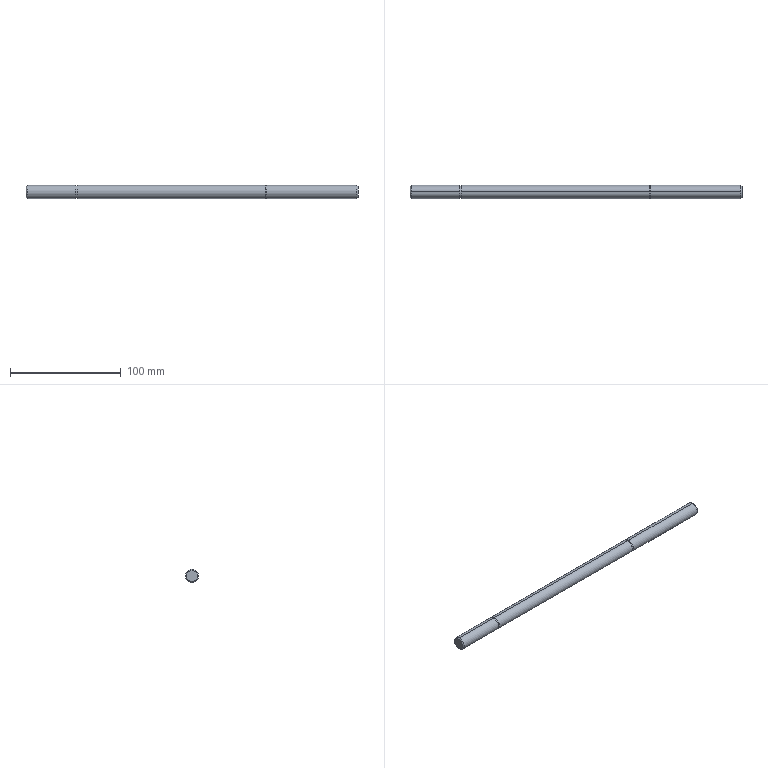Component | SolidWorks | 8TC-A15004-90-10A-2 | 1 solid | 20 faces | box 300 x 12 x 12 mm | volume 33872 mm3 | cylinder 10 | plane 6 | cone 4 | commonest cylinder face diameters 12 x6 11.5 x4 | material Hard Chrome Plated Rod
build123d program:
from build123d import *

# Parameters (mm, degrees)
SKETCH1_R           = 6
BOSS_EXTRUDE1_DEPTH = 150
CHAMFER1_SIZE       = 1
SKETCH2_W           = 0.5
SKETCH2_H           = 1.15
LPATTERN1_COUNT     = 2
LPATTERN1_PITCH     = 171.15


with BuildPart() as part:
    # Sketch1 → Boss-Extrude1 (new, symmetric)
    with BuildSketch(Plane(origin=(0, 0, 0), x_dir=(1, 0, 0), z_dir=(0, 1, 0))):
        with Locations(Location((0, 0, 0), (0, 0, 270))):
            Circle(SKETCH1_R)
    extrude(amount=BOSS_EXTRUDE1_DEPTH, both=True)

    # Chamfer1
    chamfer1_edges = [part.edges().sort_by_distance(p)[0] for p in [
        (0, -150, -6),
        (0, 150, -6),
    ]]
    chamfer(chamfer1_edges, length=CHAMFER1_SIZE)

    # Sketch2 → Cut-Revolve1 (revolve, cut)
    with BuildSketch(Plane.XY, mode=Mode.PRIVATE) as cut_revolve1_sk:
        with Locations((6, -104.425)):
            Rectangle(SKETCH2_W, SKETCH2_H)
    cut_revolve1 = revolve(cut_revolve1_sk.sketch.rotate(Axis((0, 0, 0), (0, -1, 0)), 90), axis=Axis((0, 0, 0), (0, -1, 0)), mode=Mode.SUBTRACT)

    # LPattern1: Cut-Revolve1 ×2
    with Locations(*[(0, i * LPATTERN1_PITCH, 0) for i in range(1, LPATTERN1_COUNT)]):
        add(cut_revolve1, mode=Mode.SUBTRACT)


solid = part.part

# Placed as in the assembly
solid = solid.moved(Location((-230, 332.3, -40), (0, 0, -90)))
STEP:
#1=COLOUR_RGB('',0.7922,0.8196,0.9333);
#2=FILL_AREA_STYLE_COLOUR('',#1);
#3=FILL_AREA_STYLE('',(#2));
#4=SURFACE_STYLE_FILL_AREA(#3);
#5=SURFACE_SIDE_STYLE('',(#4));
#6=SURFACE_STYLE_USAGE(.BOTH.,#5);
#7=PRESENTATION_STYLE_ASSIGNMENT((#6));
#8=CARTESIAN_POINT('',(-3.189,13.083,-1.811));
#9=VERTEX_POINT('',#8);
#10=CARTESIAN_POINT('',(-3.189,13.083,-1.339));
#11=VERTEX_POINT('',#10);
#12=CARTESIAN_POINT('',(-3.189,13.083,-1.575));
#13=DIRECTION('',(-1.,0.,-0.));
#14=DIRECTION('',(0.,0.,1.));
#15=AXIS2_PLACEMENT_3D('',#12,#13,#14);
#16=CIRCLE('',#15,0.2362);
#17=EDGE_CURVE('',#9,#11,#16,.T.);
#18=ORIENTED_EDGE('',*,*,#17,.T.);
#19=CARTESIAN_POINT('',(-6.406,13.083,-1.339));
#20=VERTEX_POINT('',#19);
#21=CARTESIAN_POINT('',(-3.15,13.083,-1.339));
#22=DIRECTION('',(-1.,0.,-0.));
#23=VECTOR('',#22,39.37);
#24=LINE('',#21,#23);
#25=EDGE_CURVE('',#11,#20,#24,.T.);
#26=ORIENTED_EDGE('',*,*,#25,.T.);
#27=CARTESIAN_POINT('',(-6.406,13.083,-1.811));
#28=VERTEX_POINT('',#27);
#29=CARTESIAN_POINT('',(-6.406,13.083,-1.575));
#30=DIRECTION('',(-1.,0.,-0.));
#31=DIRECTION('',(0.,0.,-1.));
#32=AXIS2_PLACEMENT_3D('',#29,#30,#31);
#33=CIRCLE('',#32,0.2362);
#34=EDGE_CURVE('',#28,#20,#33,.T.);
#35=ORIENTED_EDGE('',*,*,#34,.F.);
#36=CARTESIAN_POINT('',(-3.15,13.083,-1.811));
#37=DIRECTION('',(-1.,0.,-0.));
#38=VECTOR('',#37,39.37);
#39=LINE('',#36,#38);
#40=EDGE_CURVE('',#9,#28,#39,.T.);
#41=ORIENTED_EDGE('',*,*,#40,.F.);
#42=EDGE_LOOP('',(#18,#26,#35,#41));
#43=FACE_OUTER_BOUND('',#42,.T.);
#44=CARTESIAN_POINT('',(-3.15,13.083,-1.575));
#45=DIRECTION('',(-1.,0.,-0.));
#46=DIRECTION('',(0.,0.,-1.));
#47=AXIS2_PLACEMENT_3D('',#44,#45,#46);
#48=CYLINDRICAL_SURFACE('',#47,0.2362);
#49=ADVANCED_FACE('',(#43),#48,.T.);
#50=CARTESIAN_POINT('',(-3.15,13.083,-1.378));
#51=VERTEX_POINT('',#50);
#52=CARTESIAN_POINT('',(-3.15,13.083,-1.772));
#53=VERTEX_POINT('',#52);
#54=CARTESIAN_POINT('',(-3.15,13.083,-1.575));
#55=DIRECTION('',(1.,-0.,0.));
#56=DIRECTION('',(0.,0.,1.));
#57=AXIS2_PLACEMENT_3D('',#54,#55,#56);
#58=CIRCLE('',#57,0.1969);
#59=EDGE_CURVE('',#51,#53,#58,.T.);
#60=ORIENTED_EDGE('',*,*,#59,.F.);
#61=CARTESIAN_POINT('',(-3.15,13.083,-1.378));
#62=DIRECTION('',(-0.7071,-0.,0.7071));
#63=VECTOR('',#62,39.37);
#64=LINE('',#61,#63);
#65=EDGE_CURVE('',#51,#11,#64,.T.);
#66=ORIENTED_EDGE('',*,*,#65,.T.);
#67=ORIENTED_EDGE('',*,*,#17,.F.);
#68=CARTESIAN_POINT('',(-3.15,13.083,-1.772));
#69=DIRECTION('',(-0.7071,0.,-0.7071));
#70=VECTOR('',#69,39.37);
#71=LINE('',#68,#70);
#72=EDGE_CURVE('',#53,#9,#71,.T.);
#73=ORIENTED_EDGE('',*,*,#72,.F.);
#74=EDGE_LOOP('',(#60,#66,#67,#73));
#75=FACE_OUTER_BOUND('',#74,.T.);
#76=CARTESIAN_POINT('',(-3.15,13.083,-1.575));
#77=DIRECTION('',(-1.,0.,-0.));
#78=DIRECTION('',(0.,0.,-1.));
#79=AXIS2_PLACEMENT_3D('',#76,#77,#78);
#80=CONICAL_SURFACE('',#79,0.1969,0.7854);
#81=ADVANCED_FACE('',(#75),#80,.T.);
#82=CARTESIAN_POINT('',(-6.451,13.083,-1.348));
#83=VERTEX_POINT('',#82);
#84=CARTESIAN_POINT('',(-6.451,13.083,-1.801));
#85=VERTEX_POINT('',#84);
#86=CARTESIAN_POINT('',(-6.451,13.083,-1.575));
#87=DIRECTION('',(1.,-0.,0.));
#88=DIRECTION('',(0.,0.,1.));
#89=AXIS2_PLACEMENT_3D('',#86,#87,#88);
#90=CIRCLE('',#89,0.2264);
#91=EDGE_CURVE('',#83,#85,#90,.T.);
#92=ORIENTED_EDGE('',*,*,#91,.T.);
#93=CARTESIAN_POINT('',(-6.406,13.083,-1.801));
#94=VERTEX_POINT('',#93);
#95=CARTESIAN_POINT('',(-2.317,13.083,-1.801));
#96=DIRECTION('',(1.,-0.,0.));
#97=VECTOR('',#96,39.37);
#98=LINE('',#95,#97);
#99=EDGE_CURVE('',#85,#94,#98,.T.);
#100=ORIENTED_EDGE('',*,*,#99,.T.);
#101=CARTESIAN_POINT('',(-6.406,13.083,-1.348));
#102=VERTEX_POINT('',#101);
#103=CARTESIAN_POINT('',(-6.406,13.083,-1.575));
#104=DIRECTION('',(1.,-0.,0.));
#105=DIRECTION('',(0.,0.,1.));
#106=AXIS2_PLACEMENT_3D('',#103,#104,#105);
#107=CIRCLE('',#106,0.2264);
#108=EDGE_CURVE('',#102,#94,#107,.T.);
#109=ORIENTED_EDGE('',*,*,#108,.F.);
#110=CARTESIAN_POINT('',(-2.317,13.083,-1.348));
#111=DIRECTION('',(1.,-0.,0.));
#112=VECTOR('',#111,39.37);
#113=LINE('',#110,#112);
#114=EDGE_CURVE('',#83,#102,#113,.T.);
#115=ORIENTED_EDGE('',*,*,#114,.F.);
#116=EDGE_LOOP('',(#92,#100,#109,#115));
#117=FACE_OUTER_BOUND('',#116,.T.);
#118=CARTESIAN_POINT('',(-2.317,13.083,-1.575));
#119=DIRECTION('',(1.,-0.,0.));
#120=DIRECTION('',(0.,0.,1.));
#121=AXIS2_PLACEMENT_3D('',#118,#119,#120);
#122=CYLINDRICAL_SURFACE('',#121,0.2264);
#123=ADVANCED_FACE('',(#117),#122,.T.);
#124=CARTESIAN_POINT('',(-13.189,13.083,-1.339));
#125=VERTEX_POINT('',#124);
#126=CARTESIAN_POINT('',(-13.189,13.083,-1.811));
#127=VERTEX_POINT('',#126);
#128=CARTESIAN_POINT('',(-13.189,13.083,-1.575));
#129=DIRECTION('',(1.,-0.,0.));
#130=DIRECTION('',(0.,0.,1.));
#131=AXIS2_PLACEMENT_3D('',#128,#129,#130);
#132=CIRCLE('',#131,0.2362);
#133=EDGE_CURVE('',#125,#127,#132,.T.);
#134=ORIENTED_EDGE('',*,*,#133,.F.);
#135=CARTESIAN_POINT('',(-14.921,13.083,-1.339));
#136=VERTEX_POINT('',#135);
#137=CARTESIAN_POINT('',(-3.15,13.083,-1.339));
#138=DIRECTION('',(-1.,0.,-0.));
#139=VECTOR('',#138,39.37);
#140=LINE('',#137,#139);
#141=EDGE_CURVE('',#125,#136,#140,.T.);
#142=ORIENTED_EDGE('',*,*,#141,.T.);
#143=CARTESIAN_POINT('',(-14.921,13.083,-1.811));
#144=VERTEX_POINT('',#143);
#145=CARTESIAN_POINT('',(-14.921,13.083,-1.575));
#146=DIRECTION('',(1.,-0.,0.));
#147=DIRECTION('',(0.,0.,1.));
#148=AXIS2_PLACEMENT_3D('',#145,#146,#147);
#149=CIRCLE('',#148,0.2362);
#150=EDGE_CURVE('',#136,#144,#149,.T.);
#151=ORIENTED_EDGE('',*,*,#150,.T.);
#152=CARTESIAN_POINT('',(-3.15,13.083,-1.811));
#153=DIRECTION('',(-1.,0.,-0.));
#154=VECTOR('',#153,39.37);
#155=LINE('',#152,#154);
#156=EDGE_CURVE('',#127,#144,#155,.T.);
#157=ORIENTED_EDGE('',*,*,#156,.F.);
#158=EDGE_LOOP('',(#134,#142,#151,#157));
#159=FACE_OUTER_BOUND('',#158,.T.);
#160=CARTESIAN_POINT('',(-3.15,13.083,-1.575));
#161=DIRECTION('',(-1.,0.,-0.));
#162=DIRECTION('',(0.,0.,-1.));
#163=AXIS2_PLACEMENT_3D('',#160,#161,#162);
#164=CYLINDRICAL_SURFACE('',#163,0.2362);
#165=ADVANCED_FACE('',(#159),#164,.T.);
#166=CARTESIAN_POINT('',(-14.961,13.083,-1.772));
#167=VERTEX_POINT('',#166);
#168=CARTESIAN_POINT('',(-14.961,13.083,-1.378));
#169=VERTEX_POINT('',#168);
#170=CARTESIAN_POINT('',(-14.961,13.083,-1.575));
#171=DIRECTION('',(-1.,0.,-0.));
#172=DIRECTION('',(0.,0.,1.));
#173=AXIS2_PLACEMENT_3D('',#170,#171,#172);
#174=CIRCLE('',#173,0.1969);
#175=EDGE_CURVE('',#167,#169,#174,.T.);
#176=ORIENTED_EDGE('',*,*,#175,.F.);
#177=CARTESIAN_POINT('',(-14.921,13.083,-1.811));
#178=DIRECTION('',(0.7071,-0.,-0.7071));
#179=VECTOR('',#178,39.37);
#180=LINE('',#177,#179);
#181=EDGE_CURVE('',#167,#144,#180,.T.);
#182=ORIENTED_EDGE('',*,*,#181,.T.);
#183=ORIENTED_EDGE('',*,*,#150,.F.);
#184=CARTESIAN_POINT('',(-14.921,13.083,-1.339));
#185=DIRECTION('',(0.7071,-0.,0.7071));
#186=VECTOR('',#185,39.37);
#187=LINE('',#184,#186);
#188=EDGE_CURVE('',#169,#136,#187,.T.);
#189=ORIENTED_EDGE('',*,*,#188,.F.);
#190=EDGE_LOOP('',(#176,#182,#183,#189));
#191=FACE_OUTER_BOUND('',#190,.T.);
#192=CARTESIAN_POINT('',(-14.921,13.083,-1.575));
#193=DIRECTION('',(1.,-0.,0.));
#194=DIRECTION('',(0.,0.,1.));
#195=AXIS2_PLACEMENT_3D('',#192,#193,#194);
#196=CONICAL_SURFACE('',#195,0.2362,0.7854);
#197=ADVANCED_FACE('',(#191),#196,.T.);
#198=CARTESIAN_POINT('',(-13.189,13.083,-1.348));
#199=VERTEX_POINT('',#198);
#200=CARTESIAN_POINT('',(-13.189,13.083,-1.801));
#201=VERTEX_POINT('',#200);
#202=CARTESIAN_POINT('',(-13.189,13.083,-1.575));
#203=DIRECTION('',(1.,-0.,0.));
#204=DIRECTION('',(0.,0.,1.));
#205=AXIS2_PLACEMENT_3D('',#202,#203,#204);
#206=CIRCLE('',#205,0.2264);
#207=EDGE_CURVE('',#199,#201,#206,.T.);
#208=ORIENTED_EDGE('',*,*,#207,.T.);
#209=CARTESIAN_POINT('',(-13.144,13.083,-1.801));
#210=VERTEX_POINT('',#209);
#211=CARTESIAN_POINT('',(-9.055,13.083,-1.801));
#212=DIRECTION('',(1.,-0.,0.));
#213=VECTOR('',#212,39.37);
#214=LINE('',#211,#213);
#215=EDGE_CURVE('',#201,#210,#214,.T.);
#216=ORIENTED_EDGE('',*,*,#215,.T.);
#217=CARTESIAN_POINT('',(-13.144,13.083,-1.348));
#218=VERTEX_POINT('',#217);
#219=CARTESIAN_POINT('',(-13.144,13.083,-1.575));
#220=DIRECTION('',(1.,-0.,0.));
#221=DIRECTION('',(0.,0.,1.));
#222=AXIS2_PLACEMENT_3D('',#219,#220,#221);
#223=CIRCLE('',#222,0.2264);
#224=EDGE_CURVE('',#218,#210,#223,.T.);
#225=ORIENTED_EDGE('',*,*,#224,.F.);
#226=CARTESIAN_POINT('',(-9.055,13.083,-1.348));
#227=DIRECTION('',(1.,-0.,0.));
#228=VECTOR('',#227,39.37);
#229=LINE('',#226,#228);
#230=EDGE_CURVE('',#199,#218,#229,.T.);
#231=ORIENTED_EDGE('',*,*,#230,.F.);
#232=EDGE_LOOP('',(#208,#216,#225,#231));
#233=FACE_OUTER_BOUND('',#232,.T.);
#234=CARTESIAN_POINT('',(-9.055,13.083,-1.575));
#235=DIRECTION('',(1.,-0.,0.));
#236=DIRECTION('',(0.,0.,1.));
#237=AXIS2_PLACEMENT_3D('',#234,#235,#236);
#238=CYLINDRICAL_SURFACE('',#237,0.2264);
#239=ADVANCED_FACE('',(#233),#238,.T.);
#240=CARTESIAN_POINT('',(-6.451,13.083,-1.339));
#241=VERTEX_POINT('',#240);
#242=CARTESIAN_POINT('',(-6.451,13.083,-1.811));
#243=VERTEX_POINT('',#242);
#244=CARTESIAN_POINT('',(-6.451,13.083,-1.575));
#245=DIRECTION('',(1.,-0.,0.));
#246=DIRECTION('',(0.,0.,1.));
#247=AXIS2_PLACEMENT_3D('',#244,#245,#246);
#248=CIRCLE('',#247,0.2362);
#249=EDGE_CURVE('',#241,#243,#248,.T.);
#250=ORIENTED_EDGE('',*,*,#249,.F.);
#251=CARTESIAN_POINT('',(-13.144,13.083,-1.339));
#252=VERTEX_POINT('',#251);
#253=CARTESIAN_POINT('',(-3.15,13.083,-1.339));
#254=DIRECTION('',(-1.,0.,-0.));
#255=VECTOR('',#254,39.37);
#256=LINE('',#253,#255);
#257=EDGE_CURVE('',#241,#252,#256,.T.);
#258=ORIENTED_EDGE('',*,*,#257,.T.);
#259=CARTESIAN_POINT('',(-13.144,13.083,-1.811));
#260=VERTEX_POINT('',#259);
#261=CARTESIAN_POINT('',(-13.144,13.083,-1.575));
#262=DIRECTION('',(-1.,0.,-0.));
#263=DIRECTION('',(0.,0.,-1.));
#264=AXIS2_PLACEMENT_3D('',#261,#262,#263);
#265=CIRCLE('',#264,0.2362);
#266=EDGE_CURVE('',#260,#252,#265,.T.);
#267=ORIENTED_EDGE('',*,*,#266,.F.);
#268=CARTESIAN_POINT('',(-3.15,13.083,-1.811));
#269=DIRECTION('',(-1.,0.,-0.));
#270=VECTOR('',#269,39.37);
#271=LINE('',#268,#270);
#272=EDGE_CURVE('',#243,#260,#271,.T.);
#273=ORIENTED_EDGE('',*,*,#272,.F.);
#274=EDGE_LOOP('',(#250,#258,#267,#273));
#275=FACE_OUTER_BOUND('',#274,.T.);
#276=CARTESIAN_POINT('',(-3.15,13.083,-1.575));
#277=DIRECTION('',(-1.,0.,-0.));
#278=DIRECTION('',(0.,0.,-1.));
#279=AXIS2_PLACEMENT_3D('',#276,#277,#278);
#280=CYLINDRICAL_SURFACE('',#279,0.2362);
#281=ADVANCED_FACE('',(#275),#280,.T.);
#282=ORIENTED_EDGE('',*,*,#257,.F.);
#283=CARTESIAN_POINT('',(-6.451,13.083,-1.575));
#284=DIRECTION('',(1.,-0.,0.));
#285=DIRECTION('',(0.,0.,1.));
#286=AXIS2_PLACEMENT_3D('',#283,#284,#285);
#287=CIRCLE('',#286,0.2362);
#288=EDGE_CURVE('',#243,#241,#287,.T.);
#289=ORIENTED_EDGE('',*,*,#288,.F.);
#290=ORIENTED_EDGE('',*,*,#272,.T.);
#291=CARTESIAN_POINT('',(-13.144,13.083,-1.575));
#292=DIRECTION('',(-1.,0.,-0.));
#293=DIRECTION('',(0.,0.,-1.));
#294=AXIS2_PLACEMENT_3D('',#291,#292,#293);
#295=CIRCLE('',#294,0.2362);
#296=EDGE_CURVE('',#252,#260,#295,.T.);
#297=ORIENTED_EDGE('',*,*,#296,.F.);
#298=EDGE_LOOP('',(#282,#289,#290,#297));
#299=FACE_OUTER_BOUND('',#298,.T.);
#300=CARTESIAN_POINT('',(-3.15,13.083,-1.575));
#301=DIRECTION('',(-1.,0.,-0.));
#302=DIRECTION('',(0.,0.,-1.));
#303=AXIS2_PLACEMENT_3D('',#300,#301,#302);
#304=CYLINDRICAL_SURFACE('',#303,0.2362);
#305=ADVANCED_FACE('',(#299),#304,.T.);
#306=ORIENTED_EDGE('',*,*,#224,.T.);
#307=CARTESIAN_POINT('',(-13.144,13.083,-1.575));
#308=DIRECTION('',(1.,-0.,0.));
#309=DIRECTION('',(0.,0.,1.));
#310=AXIS2_PLACEMENT_3D('',#307,#308,#309);
#311=CIRCLE('',#310,0.2264);
#312=EDGE_CURVE('',#210,#218,#311,.T.);
#313=ORIENTED_EDGE('',*,*,#312,.T.);
#314=EDGE_LOOP('',(#306,#313));
#315=FACE_BOUND('',#314,.T.);
#316=ORIENTED_EDGE('',*,*,#266,.T.);
#317=ORIENTED_EDGE('',*,*,#296,.T.);
#318=EDGE_LOOP('',(#316,#317));
#319=FACE_OUTER_BOUND('',#318,.T.);
#320=CARTESIAN_POINT('',(-13.144,12.837,-1.575));
#321=DIRECTION('',(-1.,0.,-0.));
#322=DIRECTION('',(0.,0.,-1.));
#323=AXIS2_PLACEMENT_3D('',#320,#321,#322);
#324=PLANE('',#323);
#325=ADVANCED_FACE('',(#315,#319),#324,.T.);
#326=ORIENTED_EDGE('',*,*,#207,.F.);
#327=CARTESIAN_POINT('',(-13.189,13.083,-1.575));
#328=DIRECTION('',(1.,-0.,0.));
#329=DIRECTION('',(0.,0.,1.));
#330=AXIS2_PLACEMENT_3D('',#327,#328,#329);
#331=CIRCLE('',#330,0.2264);
#332=EDGE_CURVE('',#201,#199,#331,.T.);
#333=ORIENTED_EDGE('',*,*,#332,.F.);
#334=EDGE_LOOP('',(#326,#333));
#335=FACE_BOUND('',#334,.T.);
#336=CARTESIAN_POINT('',(-13.189,13.083,-1.575));
#337=DIRECTION('',(1.,-0.,0.));
#338=DIRECTION('',(0.,0.,1.));
#339=AXIS2_PLACEMENT_3D('',#336,#337,#338);
#340=CIRCLE('',#339,0.2362);
#341=EDGE_CURVE('',#127,#125,#340,.T.);
#342=ORIENTED_EDGE('',*,*,#341,.T.);
#343=ORIENTED_EDGE('',*,*,#133,.T.);
#344=EDGE_LOOP('',(#342,#343));
#345=FACE_OUTER_BOUND('',#344,.T.);
#346=CARTESIAN_POINT('',(-13.189,12.837,-1.575));
#347=DIRECTION('',(1.,-0.,0.));
#348=DIRECTION('',(-0.,-0.,1.));
#349=AXIS2_PLACEMENT_3D('',#346,#347,#348);
#350=PLANE('',#349);
#351=ADVANCED_FACE('',(#335,#345),#350,.T.);
#352=ORIENTED_EDGE('',*,*,#215,.F.);
#353=ORIENTED_EDGE('',*,*,#332,.T.);
#354=ORIENTED_EDGE('',*,*,#230,.T.);
#355=ORIENTED_EDGE('',*,*,#312,.F.);
#356=EDGE_LOOP('',(#352,#353,#354,#355));
#357=FACE_OUTER_BOUND('',#356,.T.);
#358=CARTESIAN_POINT('',(-9.055,13.083,-1.575));
#359=DIRECTION('',(1.,-0.,0.));
#360=DIRECTION('',(0.,0.,1.));
#361=AXIS2_PLACEMENT_3D('',#358,#359,#360);
#362=CYLINDRICAL_SURFACE('',#361,0.2264);
#363=ADVANCED_FACE('',(#357),#362,.T.);
#364=CARTESIAN_POINT('',(-14.961,13.083,-1.575));
#365=DIRECTION('',(-1.,0.,-0.));
#366=DIRECTION('',(0.,0.,1.));
#367=AXIS2_PLACEMENT_3D('',#364,#365,#366);
#368=CIRCLE('',#367,0.1969);
#369=EDGE_CURVE('',#169,#167,#368,.T.);
#370=ORIENTED_EDGE('',*,*,#369,.T.);
#371=ORIENTED_EDGE('',*,*,#175,.T.);
#372=EDGE_LOOP('',(#370,#371));
#373=FACE_OUTER_BOUND('',#372,.T.);
#374=CARTESIAN_POINT('',(-14.961,13.083,-1.575));
#375=DIRECTION('',(1.,-0.,0.));
#376=DIRECTION('',(-0.,-0.,1.));
#377=AXIS2_PLACEMENT_3D('',#374,#375,#376);
#378=PLANE('',#377);
#379=ADVANCED_FACE('',(#373),#378,.F.);
#380=ORIENTED_EDGE('',*,*,#181,.F.);
#381=ORIENTED_EDGE('',*,*,#369,.F.);
#382=ORIENTED_EDGE('',*,*,#188,.T.);
#383=CARTESIAN_POINT('',(-14.921,13.083,-1.575));
#384=DIRECTION('',(1.,-0.,0.));
#385=DIRECTION('',(0.,0.,1.));
#386=AXIS2_PLACEMENT_3D('',#383,#384,#385);
#387=CIRCLE('',#386,0.2362);
#388=EDGE_CURVE('',#144,#136,#387,.T.);
#389=ORIENTED_EDGE('',*,*,#388,.F.);
#390=EDGE_LOOP('',(#380,#381,#382,#389));
#391=FACE_OUTER_BOUND('',#390,.T.);
#392=CARTESIAN_POINT('',(-14.921,13.083,-1.575));
#393=DIRECTION('',(1.,-0.,0.));
#394=DIRECTION('',(0.,0.,1.));
#395=AXIS2_PLACEMENT_3D('',#392,#393,#394);
#396=CONICAL_SURFACE('',#395,0.2362,0.7854);
#397=ADVANCED_FACE('',(#391),#396,.T.);
#398=ORIENTED_EDGE('',*,*,#141,.F.);
#399=ORIENTED_EDGE('',*,*,#341,.F.);
#400=ORIENTED_EDGE('',*,*,#156,.T.);
#401=ORIENTED_EDGE('',*,*,#388,.T.);
#402=EDGE_LOOP('',(#398,#399,#400,#401));
#403=FACE_OUTER_BOUND('',#402,.T.);
#404=CARTESIAN_POINT('',(-3.15,13.083,-1.575));
#405=DIRECTION('',(-1.,0.,-0.));
#406=DIRECTION('',(0.,0.,-1.));
#407=AXIS2_PLACEMENT_3D('',#404,#405,#406);
#408=CYLINDRICAL_SURFACE('',#407,0.2362);
#409=ADVANCED_FACE('',(#403),#408,.T.);
#410=ORIENTED_EDGE('',*,*,#108,.T.);
#411=CARTESIAN_POINT('',(-6.406,13.083,-1.575));
#412=DIRECTION('',(1.,-0.,0.));
#413=DIRECTION('',(0.,0.,1.));
#414=AXIS2_PLACEMENT_3D('',#411,#412,#413);
#415=CIRCLE('',#414,0.2264);
#416=EDGE_CURVE('',#94,#102,#415,.T.);
#417=ORIENTED_EDGE('',*,*,#416,.T.);
#418=EDGE_LOOP('',(#410,#417));
#419=FACE_BOUND('',#418,.T.);
#420=ORIENTED_EDGE('',*,*,#34,.T.);
#421=CARTESIAN_POINT('',(-6.406,13.083,-1.575));
#422=DIRECTION('',(-1.,0.,-0.));
#423=DIRECTION('',(0.,0.,-1.));
#424=AXIS2_PLACEMENT_3D('',#421,#422,#423);
#425=CIRCLE('',#424,0.2362);
#426=EDGE_CURVE('',#20,#28,#425,.T.);
#427=ORIENTED_EDGE('',*,*,#426,.T.);
#428=EDGE_LOOP('',(#420,#427));
#429=FACE_OUTER_BOUND('',#428,.T.);
#430=CARTESIAN_POINT('',(-6.406,12.837,-1.575));
#431=DIRECTION('',(-1.,0.,-0.));
#432=DIRECTION('',(0.,0.,-1.));
#433=AXIS2_PLACEMENT_3D('',#430,#431,#432);
#434=PLANE('',#433);
#435=ADVANCED_FACE('',(#419,#429),#434,.T.);
#436=ORIENTED_EDGE('',*,*,#91,.F.);
#437=CARTESIAN_POINT('',(-6.451,13.083,-1.575));
#438=DIRECTION('',(1.,-0.,0.));
#439=DIRECTION('',(0.,0.,1.));
#440=AXIS2_PLACEMENT_3D('',#437,#438,#439);
#441=CIRCLE('',#440,0.2264);
#442=EDGE_CURVE('',#85,#83,#441,.T.);
#443=ORIENTED_EDGE('',*,*,#442,.F.);
#444=EDGE_LOOP('',(#436,#443));
#445=FACE_BOUND('',#444,.T.);
#446=ORIENTED_EDGE('',*,*,#288,.T.);
#447=ORIENTED_EDGE('',*,*,#249,.T.);
#448=EDGE_LOOP('',(#446,#447));
#449=FACE_OUTER_BOUND('',#448,.T.);
#450=CARTESIAN_POINT('',(-6.451,12.837,-1.575));
#451=DIRECTION('',(1.,-0.,0.));
#452=DIRECTION('',(-0.,-0.,1.));
#453=AXIS2_PLACEMENT_3D('',#450,#451,#452);
#454=PLANE('',#453);
#455=ADVANCED_FACE('',(#445,#449),#454,.T.);
#456=ORIENTED_EDGE('',*,*,#99,.F.);
#457=ORIENTED_EDGE('',*,*,#442,.T.);
#458=ORIENTED_EDGE('',*,*,#114,.T.);
#459=ORIENTED_EDGE('',*,*,#416,.F.);
#460=EDGE_LOOP('',(#456,#457,#458,#459));
#461=FACE_OUTER_BOUND('',#460,.T.);
#462=CARTESIAN_POINT('',(-2.317,13.083,-1.575));
#463=DIRECTION('',(1.,-0.,0.));
#464=DIRECTION('',(0.,0.,1.));
#465=AXIS2_PLACEMENT_3D('',#462,#463,#464);
#466=CYLINDRICAL_SURFACE('',#465,0.2264);
#467=ADVANCED_FACE('',(#461),#466,.T.);
#468=CARTESIAN_POINT('',(-3.15,13.083,-1.575));
#469=DIRECTION('',(1.,-0.,0.));
#470=DIRECTION('',(0.,0.,1.));
#471=AXIS2_PLACEMENT_3D('',#468,#469,#470);
#472=CIRCLE('',#471,0.1969);
#473=EDGE_CURVE('',#53,#51,#472,.T.);
#474=ORIENTED_EDGE('',*,*,#473,.T.);
#475=ORIENTED_EDGE('',*,*,#59,.T.);
#476=EDGE_LOOP('',(#474,#475));
#477=FACE_OUTER_BOUND('',#476,.T.);
#478=CARTESIAN_POINT('',(-3.15,13.083,-1.575));
#479=DIRECTION('',(1.,-0.,0.));
#480=DIRECTION('',(-0.,-0.,1.));
#481=AXIS2_PLACEMENT_3D('',#478,#479,#480);
#482=PLANE('',#481);
#483=ADVANCED_FACE('',(#477),#482,.T.);
#484=ORIENTED_EDGE('',*,*,#65,.F.);
#485=ORIENTED_EDGE('',*,*,#473,.F.);
#486=ORIENTED_EDGE('',*,*,#72,.T.);
#487=CARTESIAN_POINT('',(-3.189,13.083,-1.575));
#488=DIRECTION('',(-1.,0.,-0.));
#489=DIRECTION('',(0.,0.,1.));
#490=AXIS2_PLACEMENT_3D('',#487,#488,#489);
#491=CIRCLE('',#490,0.2362);
#492=EDGE_CURVE('',#11,#9,#491,.T.);
#493=ORIENTED_EDGE('',*,*,#492,.F.);
#494=EDGE_LOOP('',(#484,#485,#486,#493));
#495=FACE_OUTER_BOUND('',#494,.T.);
#496=CARTESIAN_POINT('',(-3.15,13.083,-1.575));
#497=DIRECTION('',(-1.,0.,-0.));
#498=DIRECTION('',(0.,0.,-1.));
#499=AXIS2_PLACEMENT_3D('',#496,#497,#498);
#500=CONICAL_SURFACE('',#499,0.1969,0.7854);
#501=ADVANCED_FACE('',(#495),#500,.T.);
#502=ORIENTED_EDGE('',*,*,#25,.F.);
#503=ORIENTED_EDGE('',*,*,#492,.T.);
#504=ORIENTED_EDGE('',*,*,#40,.T.);
#505=ORIENTED_EDGE('',*,*,#426,.F.);
#506=EDGE_LOOP('',(#502,#503,#504,#505));
#507=FACE_OUTER_BOUND('',#506,.T.);
#508=CARTESIAN_POINT('',(-3.15,13.083,-1.575));
#509=DIRECTION('',(-1.,0.,-0.));
#510=DIRECTION('',(0.,0.,-1.));
#511=AXIS2_PLACEMENT_3D('',#508,#509,#510);
#512=CYLINDRICAL_SURFACE('',#511,0.2362);
#513=ADVANCED_FACE('',(#507),#512,.T.);
#514=CLOSED_SHELL('',(#49,#81,#123,#165,#197,#239,#281,#305,#325,#351,#363,#379,#397,#409,#435,#455,#467,#483,#501,#513));
#515=MANIFOLD_SOLID_BREP('',#514);
#516=STYLED_ITEM('',(#7),#515);
#517=(LENGTH_UNIT()NAMED_UNIT(*)SI_UNIT($,.METRE.));
#518=LENGTH_MEASURE_WITH_UNIT(LENGTH_MEASURE(0.0254),#517);
#519=DIMENSIONAL_EXPONENTS(1.,0.,0.,0.,0.,0.,0.);
#520=(CONVERSION_BASED_UNIT('',#518)LENGTH_UNIT()NAMED_UNIT(#519));
#521=UNCERTAINTY_MEASURE_WITH_UNIT(LENGTH_MEASURE(0.00001),#520,'','');
#522=(NAMED_UNIT(*)PLANE_ANGLE_UNIT()SI_UNIT($,.RADIAN.));
#523=(NAMED_UNIT(*)SI_UNIT($,.STERADIAN.)SOLID_ANGLE_UNIT());
#524=(GEOMETRIC_REPRESENTATION_CONTEXT(3)GLOBAL_UNCERTAINTY_ASSIGNED_CONTEXT((#521))GLOBAL_UNIT_ASSIGNED_CONTEXT((#520,#522,#523))REPRESENTATION_CONTEXT('',''));
#525=MECHANICAL_DESIGN_GEOMETRIC_PRESENTATION_REPRESENTATION('',(#516),#524);
#526=CARTESIAN_POINT('',(0.,0.,0.));
#527=DIRECTION('',(0.,0.,1.));
#528=DIRECTION('',(1.,0.,0.));
#529=AXIS2_PLACEMENT_3D('',#526,#527,#528);
#530=(LENGTH_UNIT()NAMED_UNIT(*)SI_UNIT($,.METRE.));
#531=LENGTH_MEASURE_WITH_UNIT(LENGTH_MEASURE(0.0254),#530);
#532=DIMENSIONAL_EXPONENTS(1.,0.,0.,0.,0.,0.,0.);
#533=(CONVERSION_BASED_UNIT('',#531)LENGTH_UNIT()NAMED_UNIT(#532));
#534=UNCERTAINTY_MEASURE_WITH_UNIT(LENGTH_MEASURE(0.00001),#533,'','');
#535=(NAMED_UNIT(*)PLANE_ANGLE_UNIT()SI_UNIT($,.RADIAN.));
#536=(NAMED_UNIT(*)SI_UNIT($,.STERADIAN.)SOLID_ANGLE_UNIT());
#537=(GEOMETRIC_REPRESENTATION_CONTEXT(3)GLOBAL_UNCERTAINTY_ASSIGNED_CONTEXT((#534))GLOBAL_UNIT_ASSIGNED_CONTEXT((#533,#535,#536))REPRESENTATION_CONTEXT('',''));
#538=ADVANCED_BREP_SHAPE_REPRESENTATION('',(#515,#529),#537);
#539=PRESENTATION_LAYER_ASSIGNMENT('','',(#516));